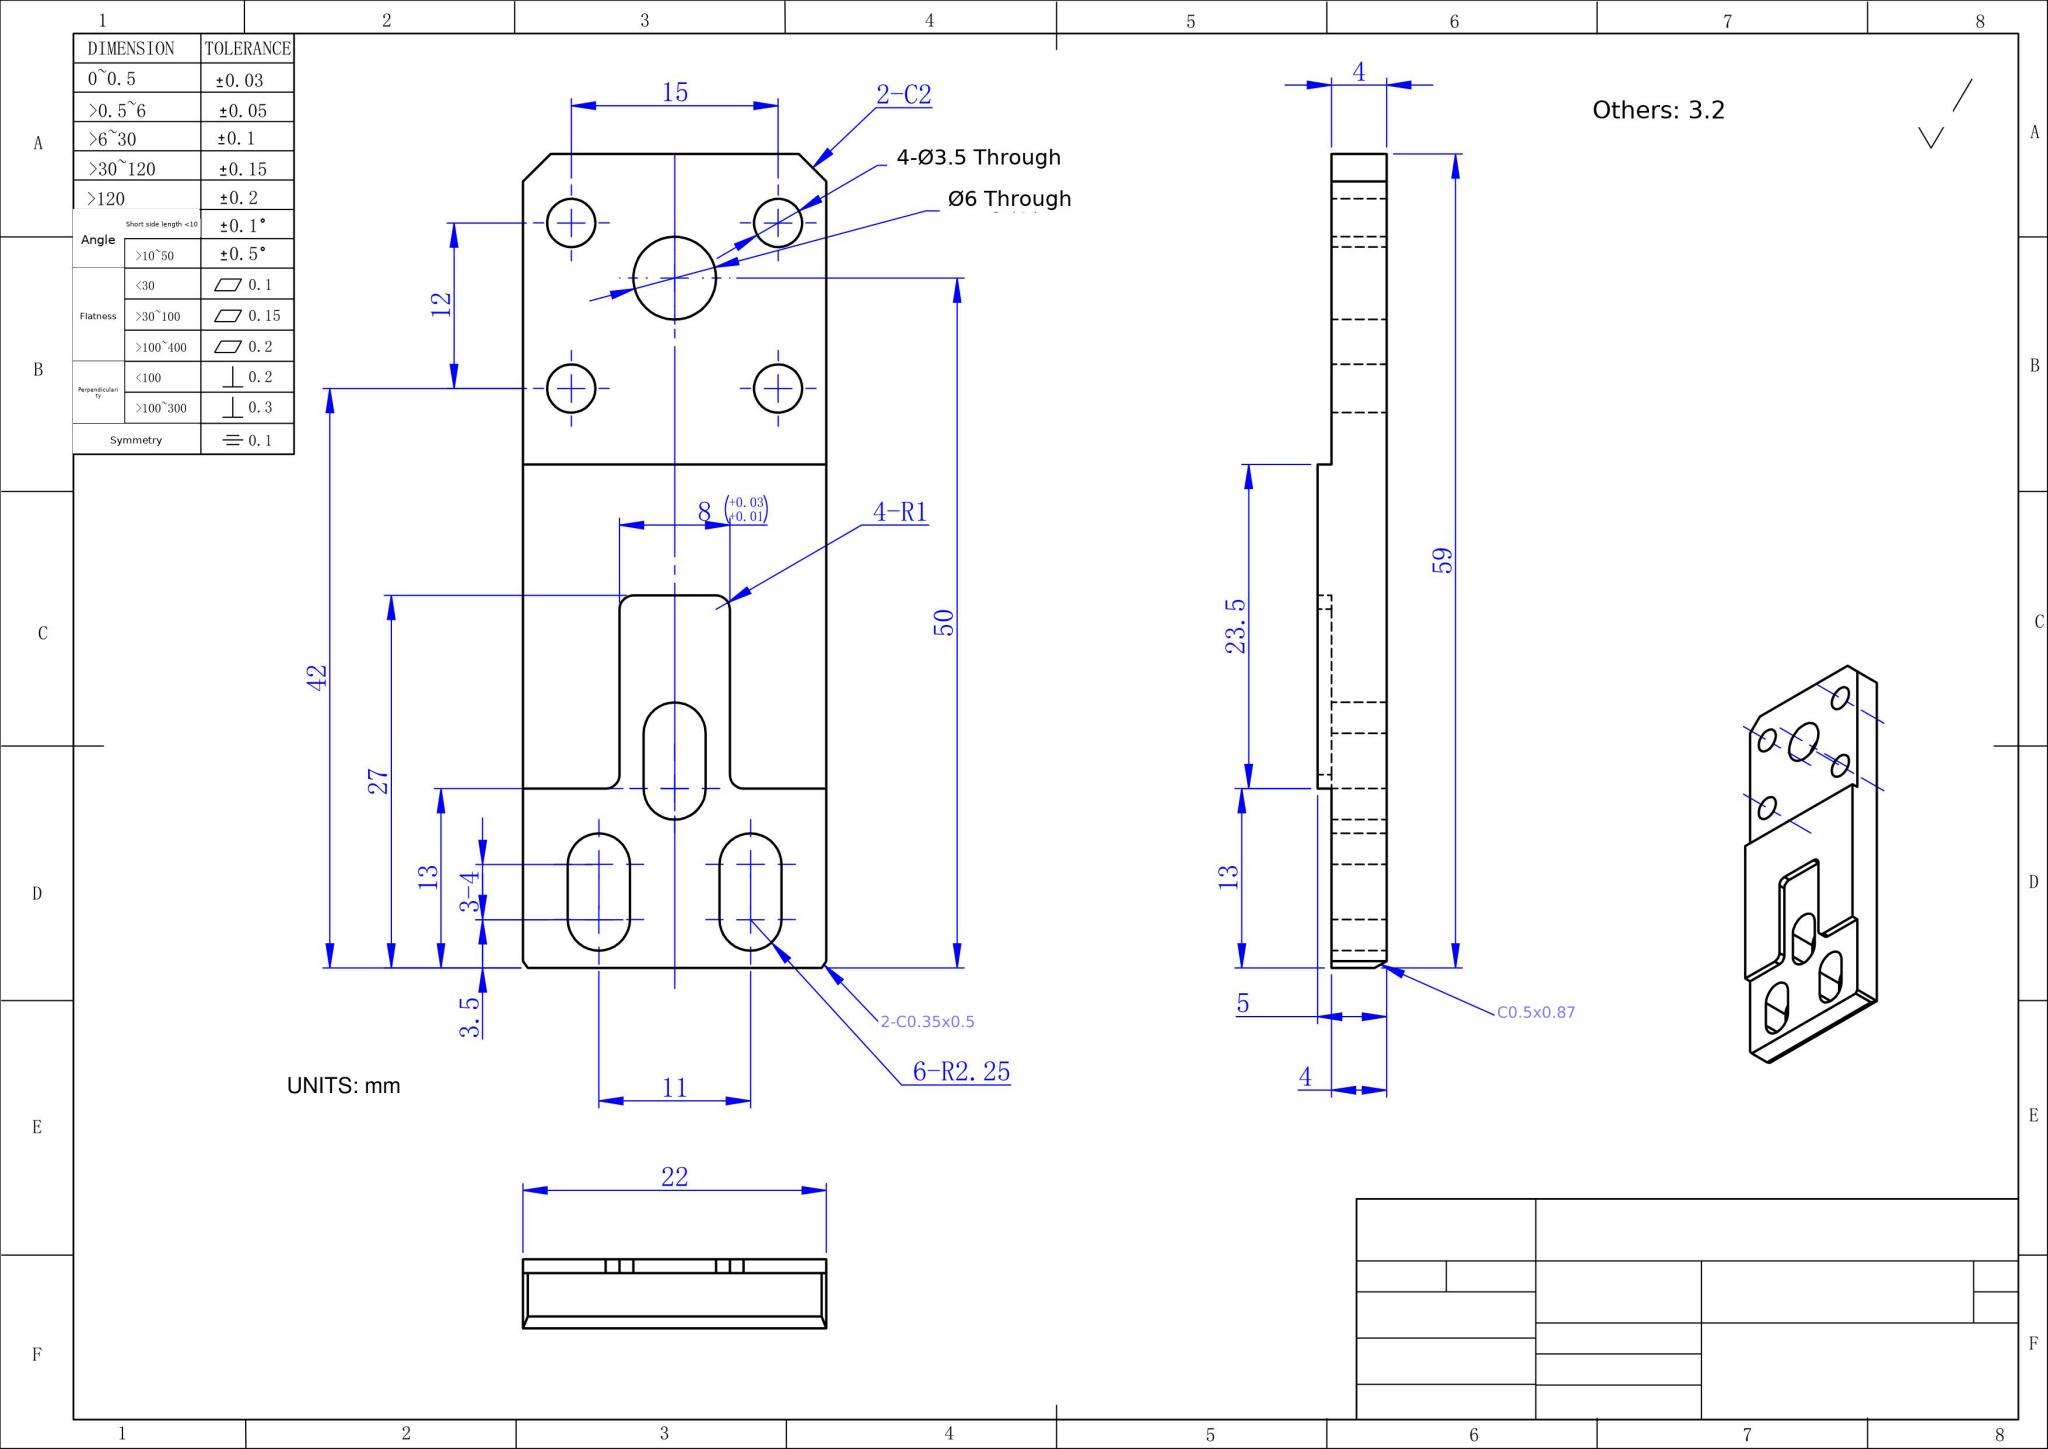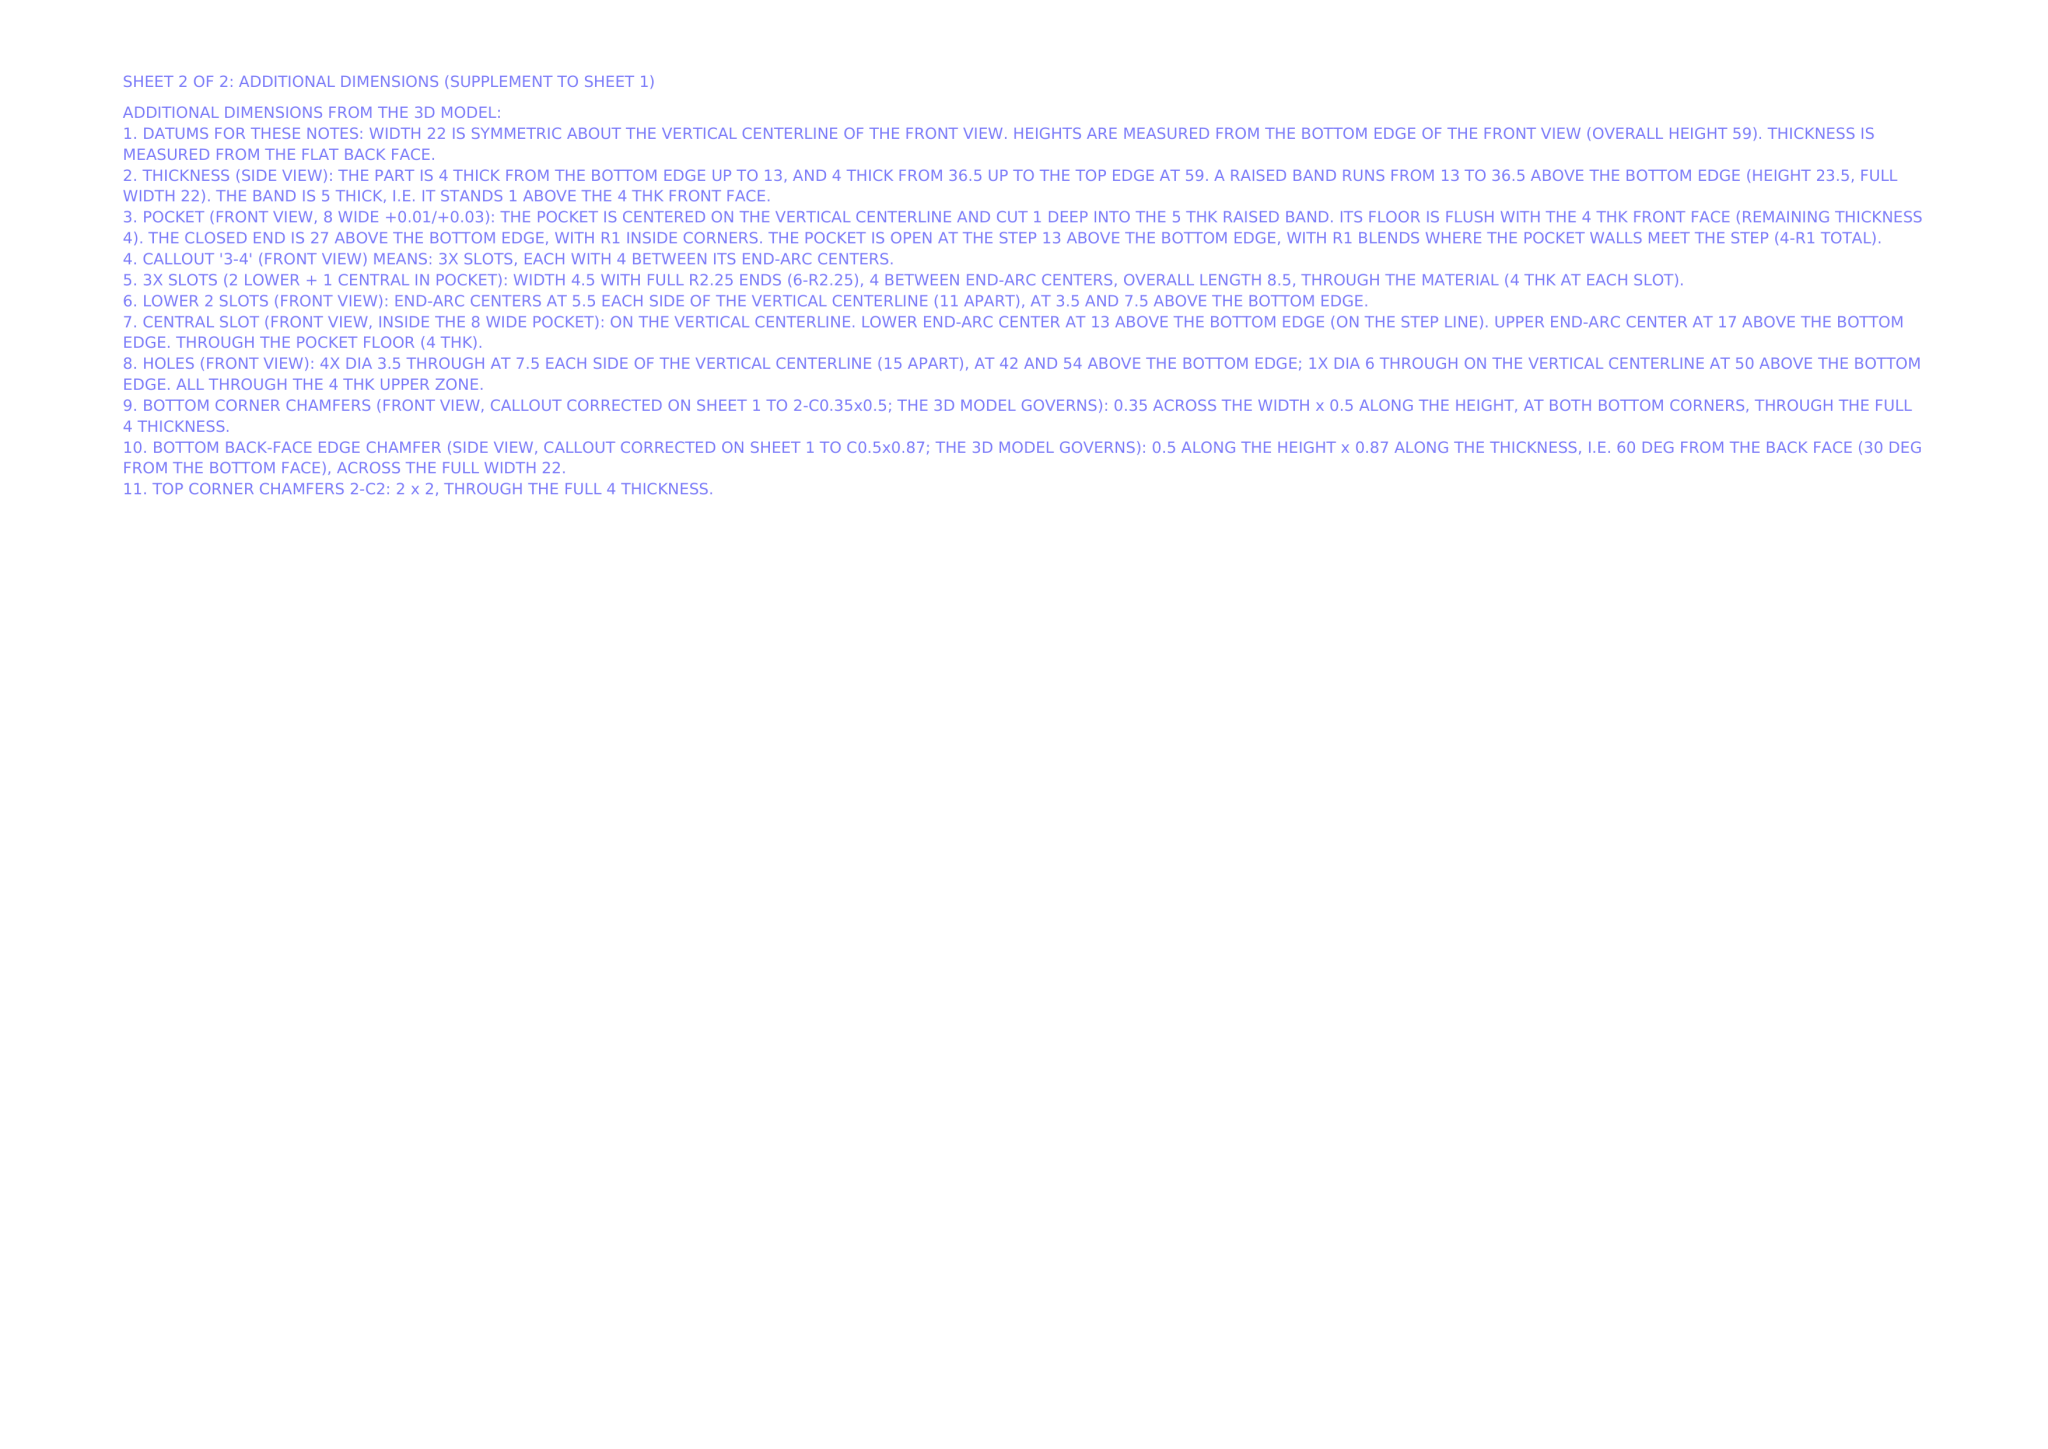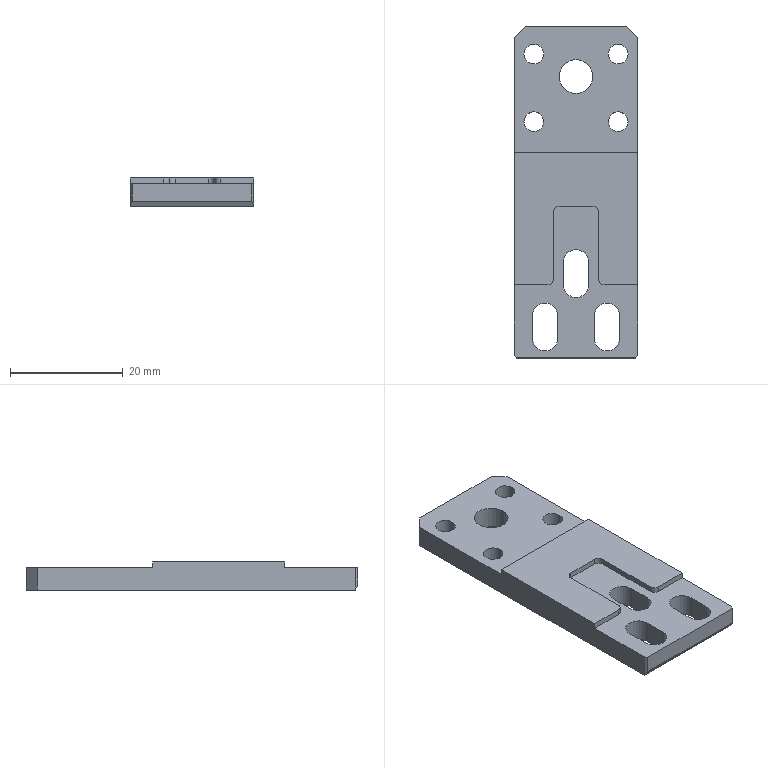Part | NX | mm | 1 solid | 45 faces | box 22 x 59 x 5 mm | volume 4902 mm3 | plane 25 | cylinder 20 | commonest cylinder face diameters 3.5 x8 4.5 x6 2 x4 6 x2